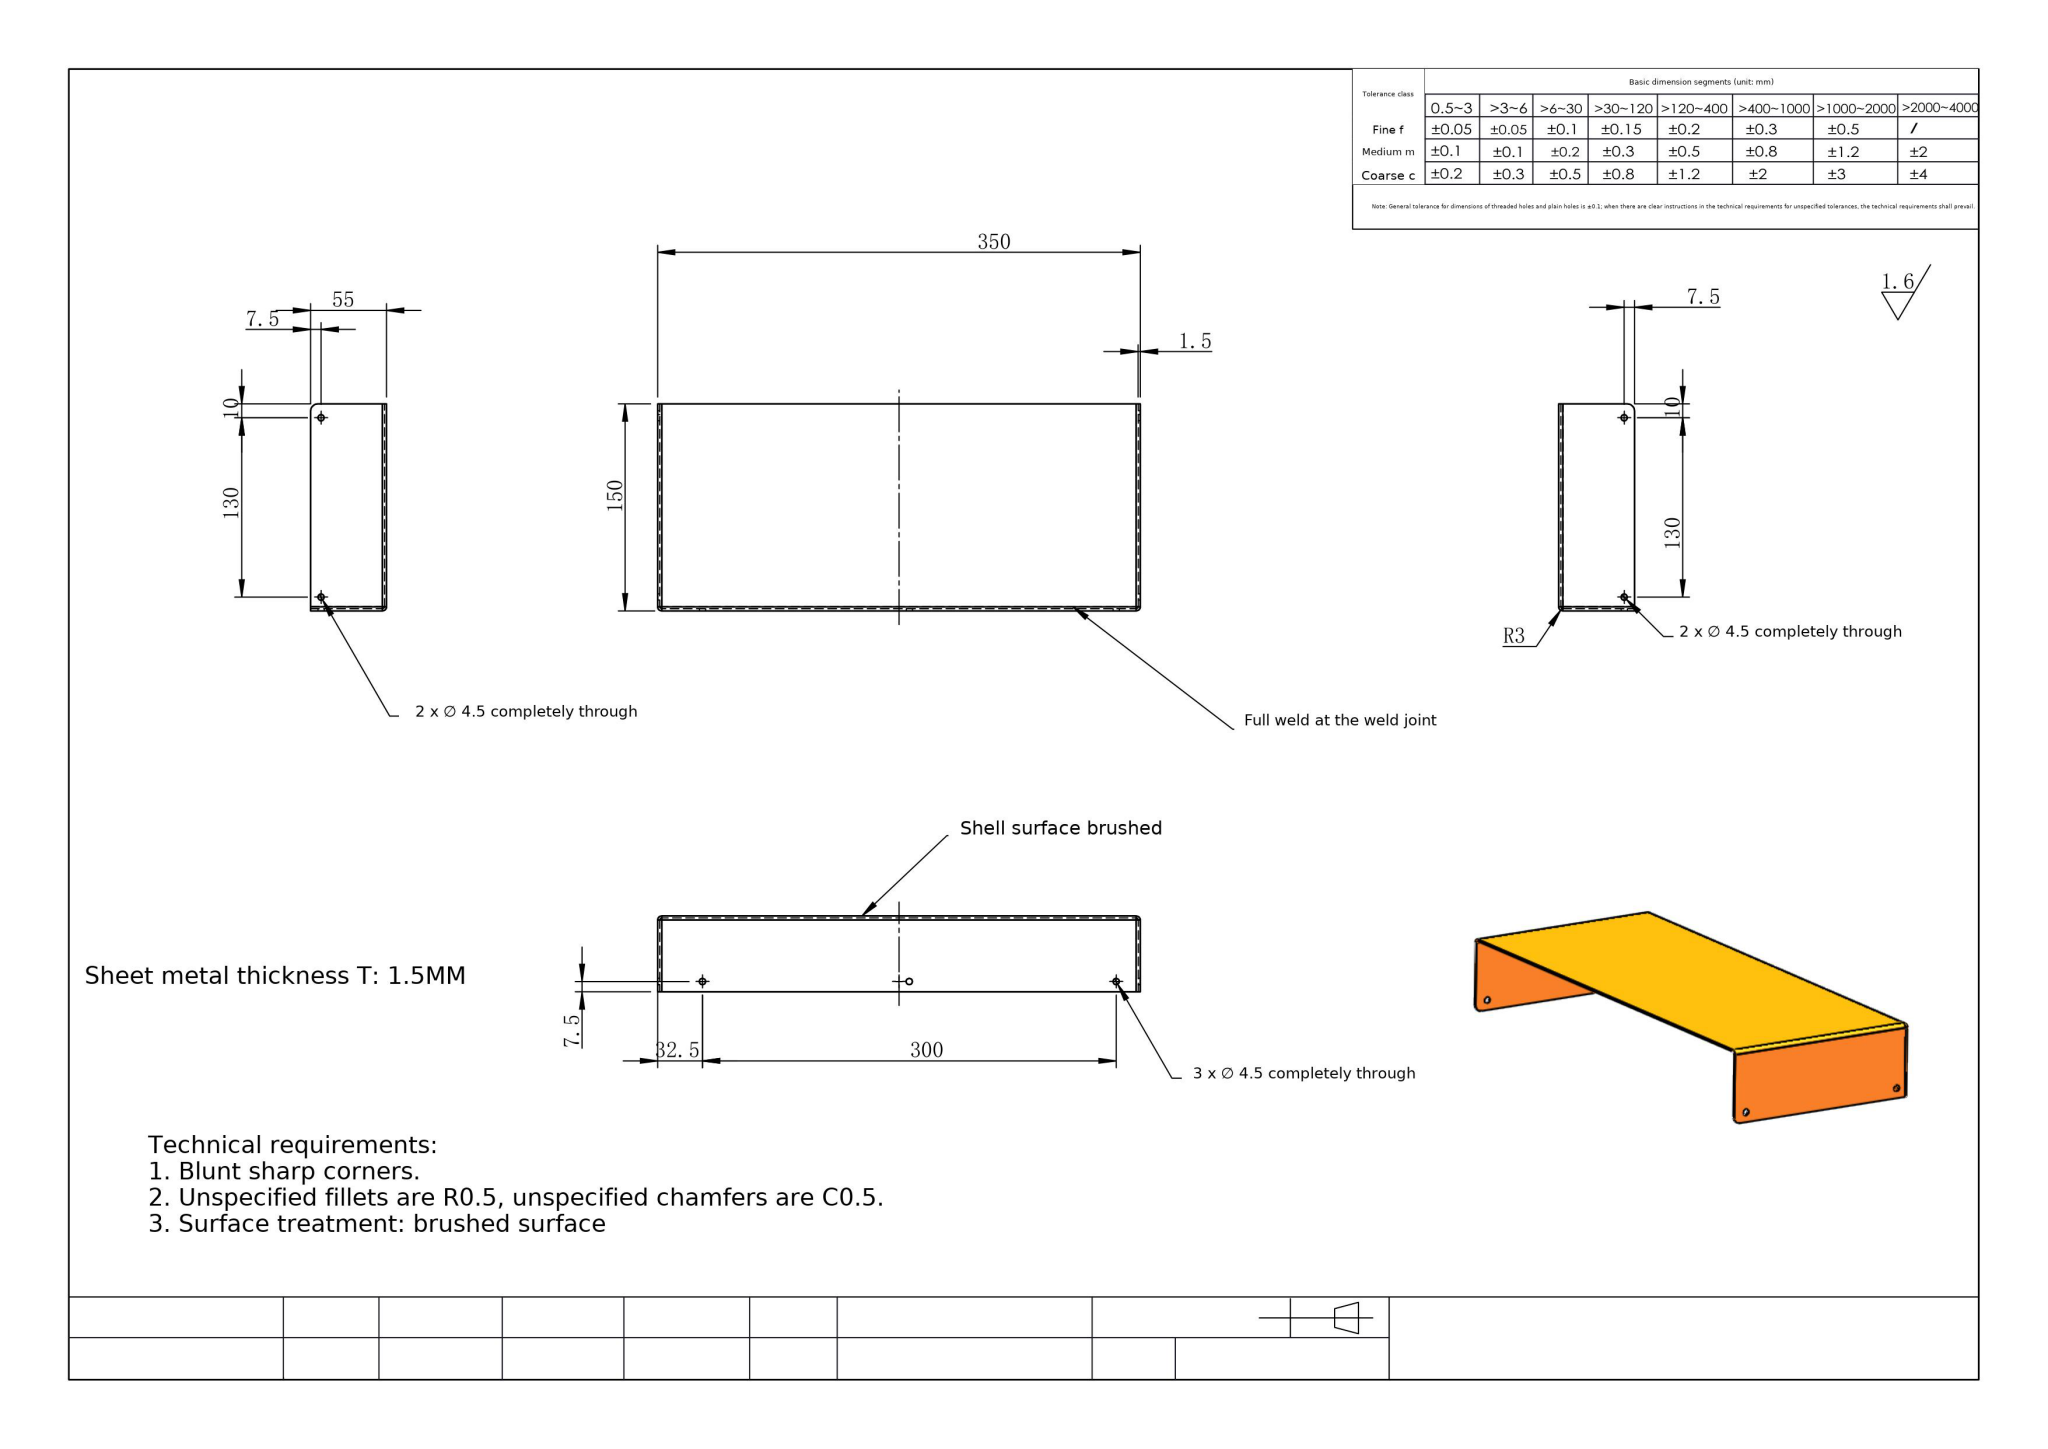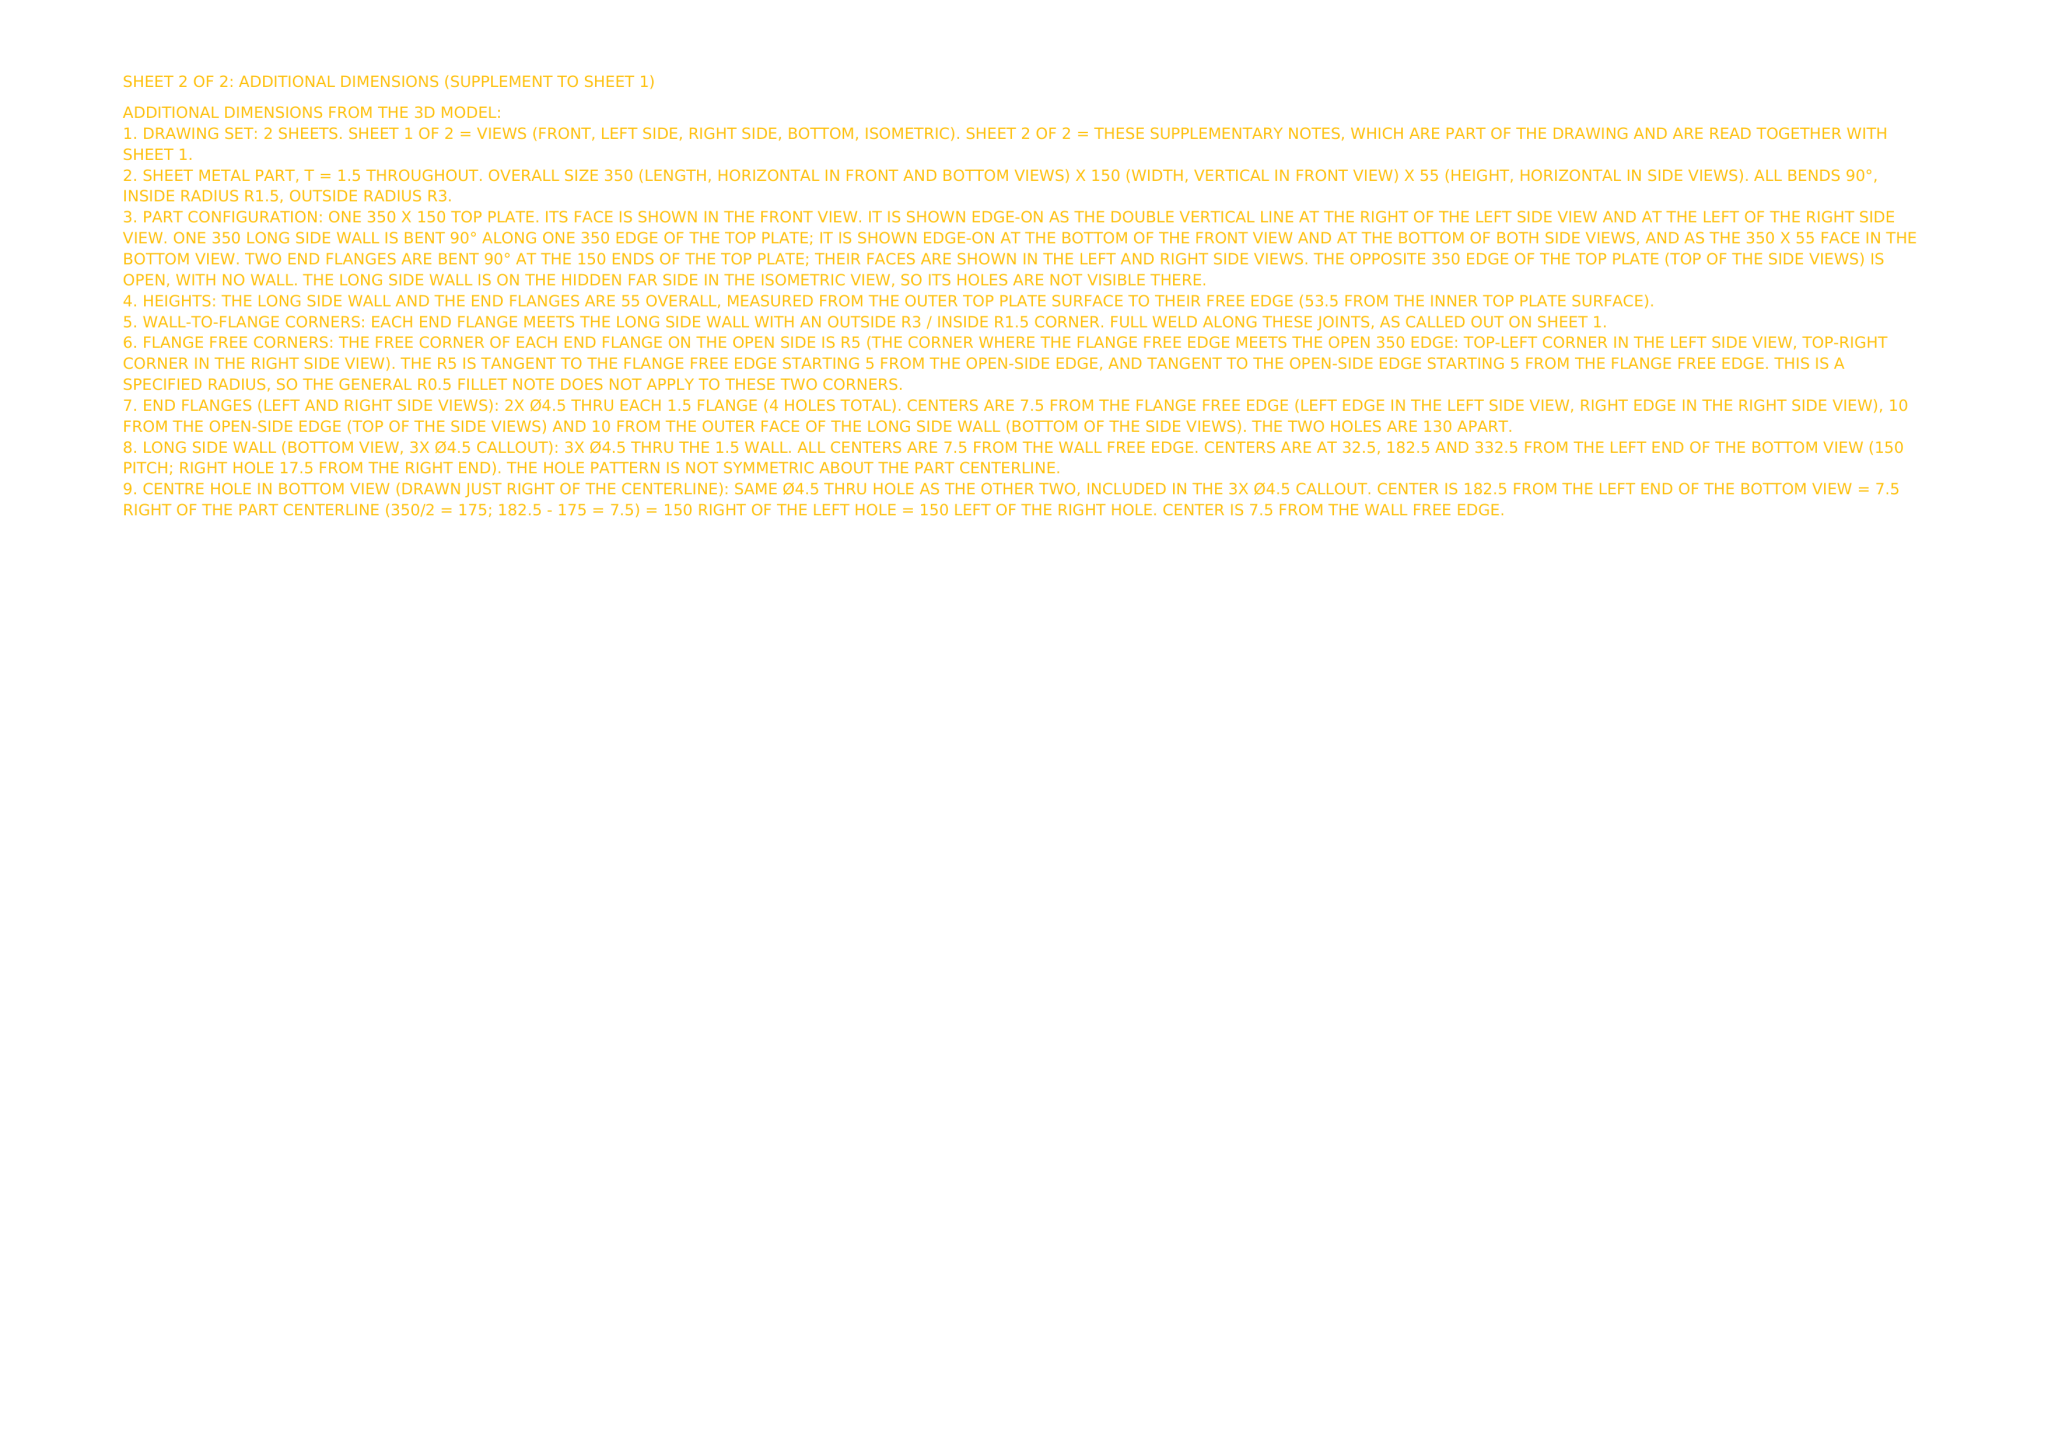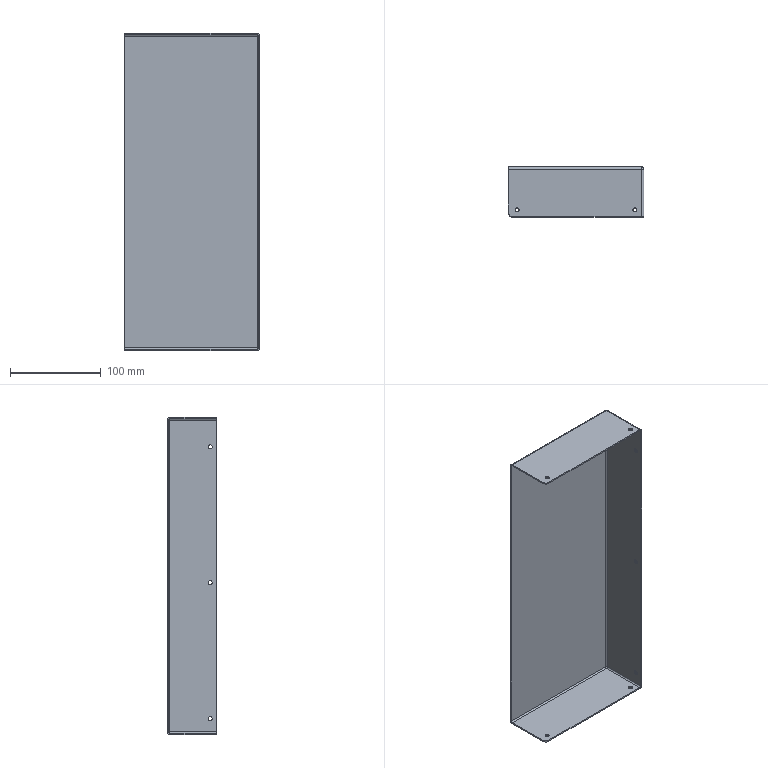Part | NX | mm | 1 solid | 40 faces | box 150 x 55 x 350 mm | volume 129391 mm3 | cylinder 26 | plane 10 | sphere 4 | commonest cylinder face diameters 4.5 x14 6 x5 3 x5 10 x2